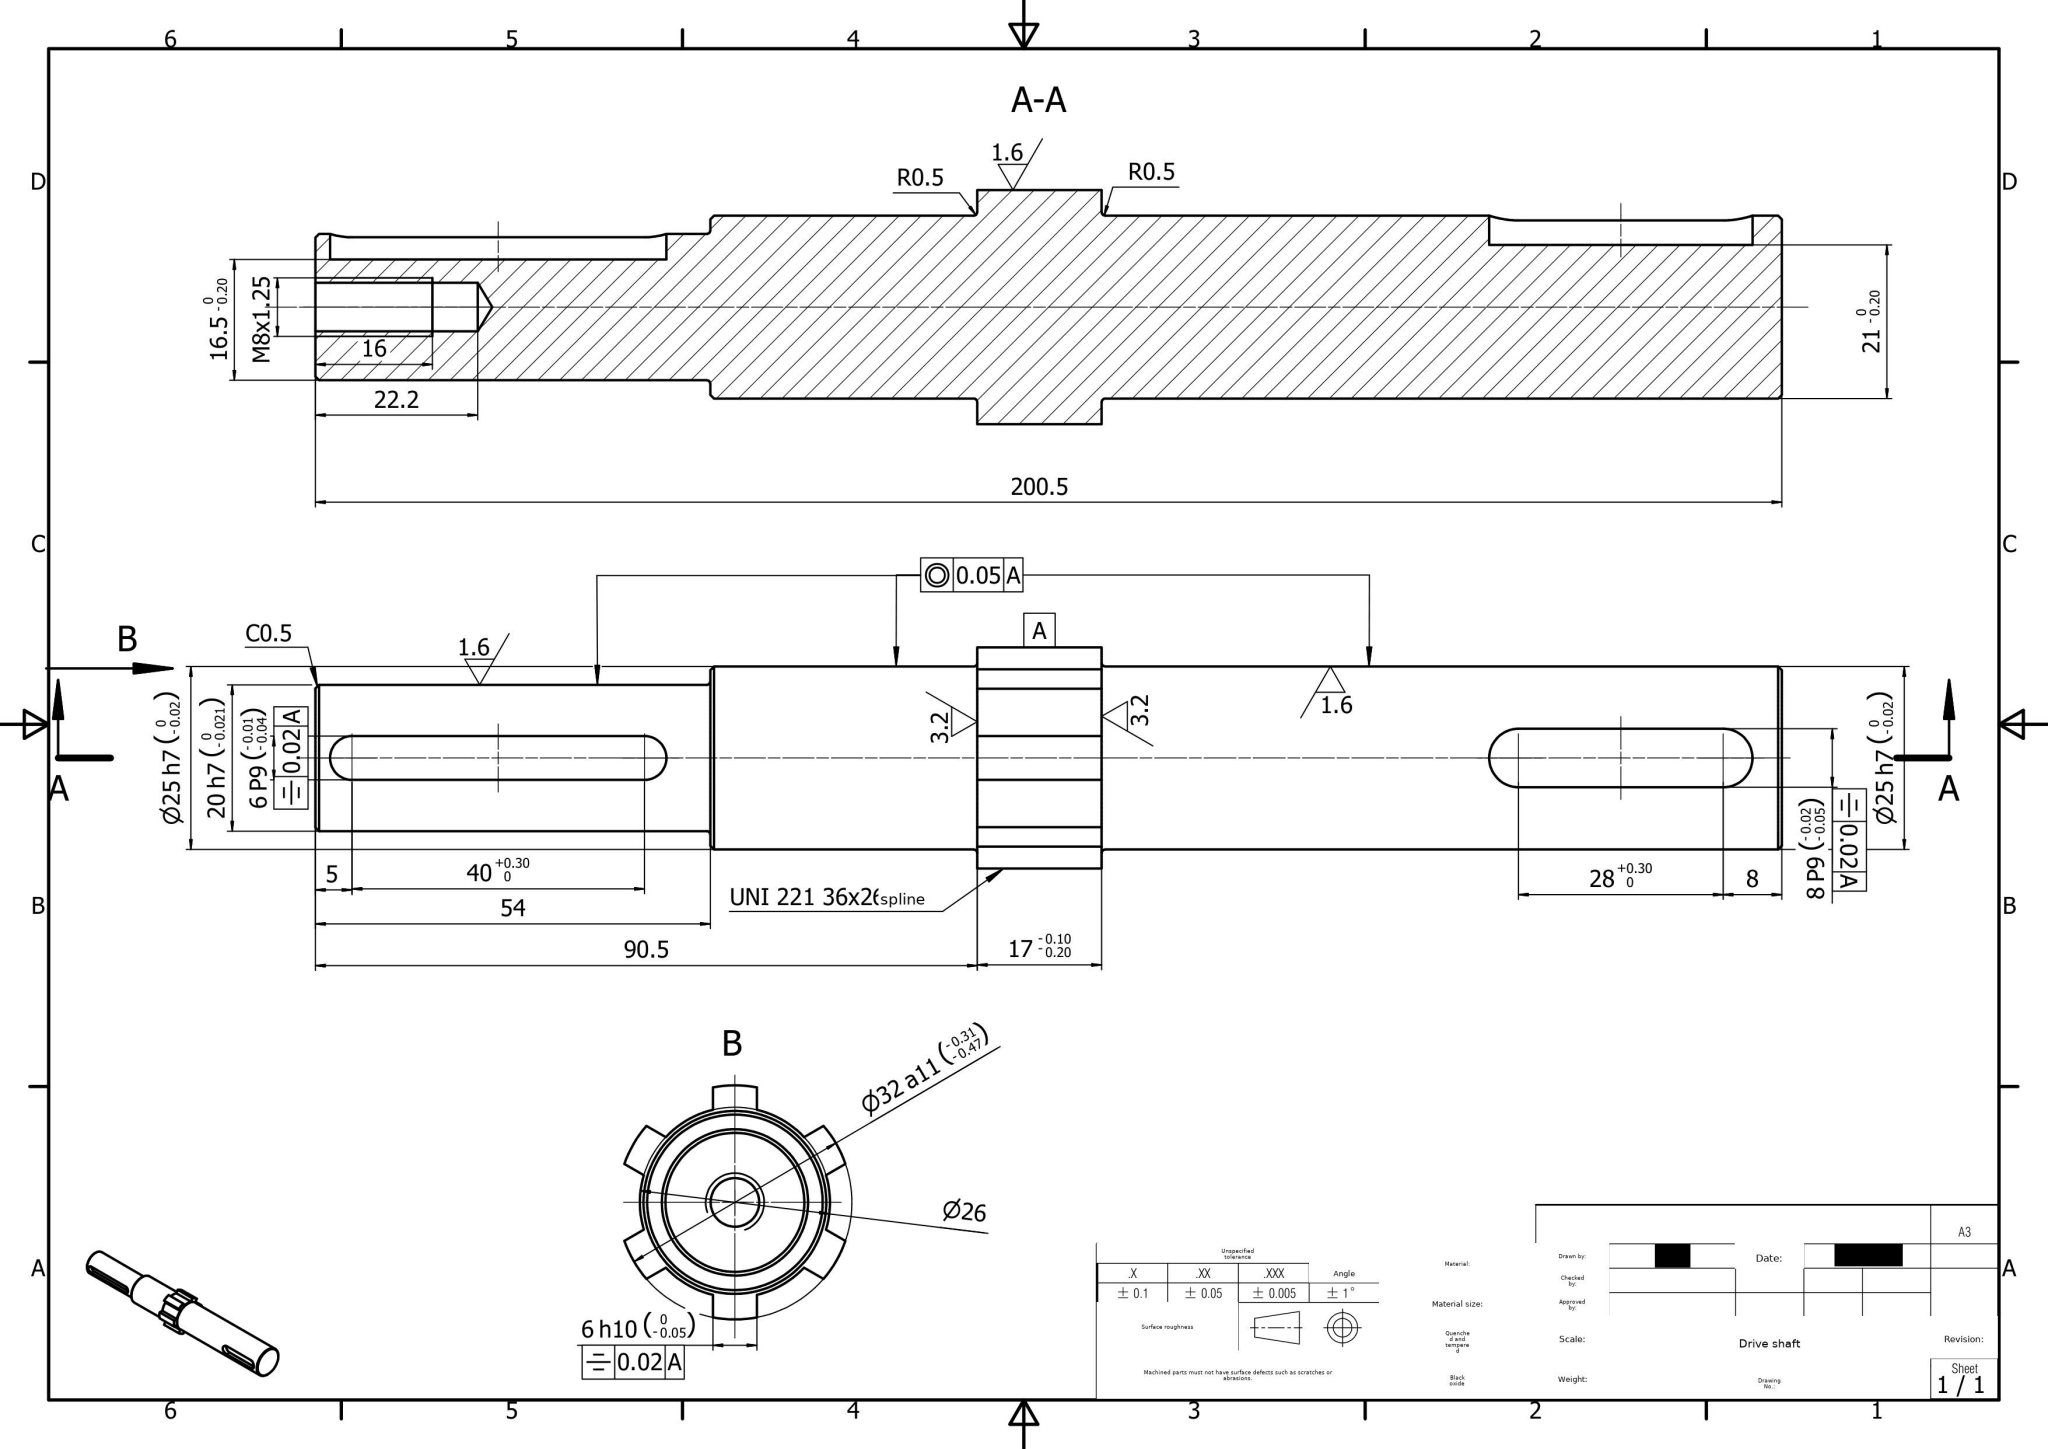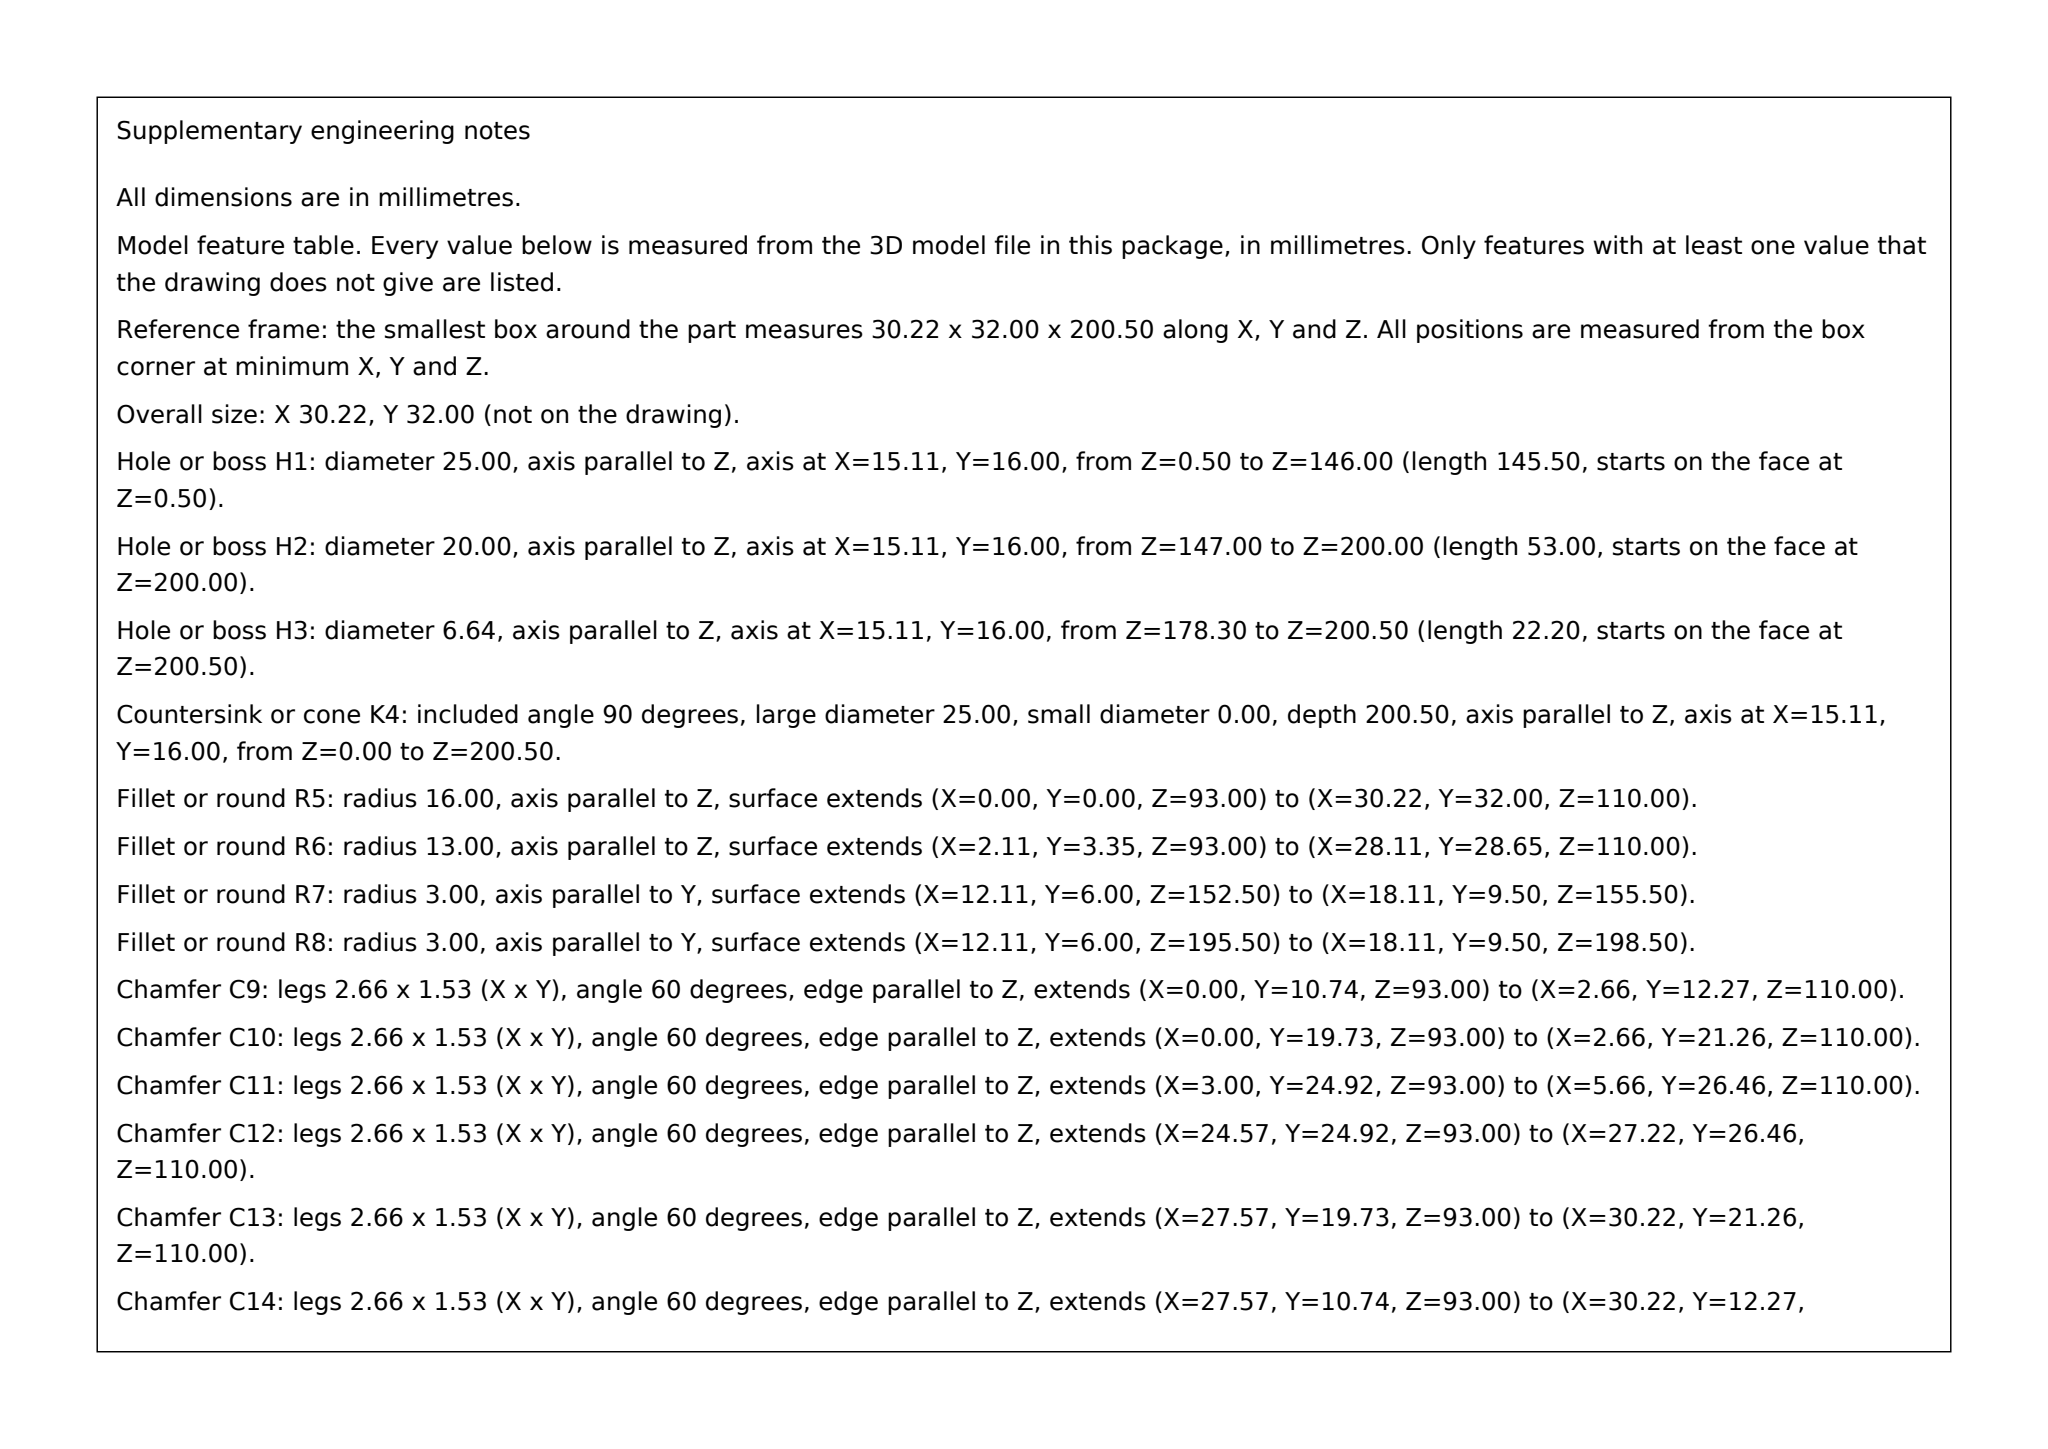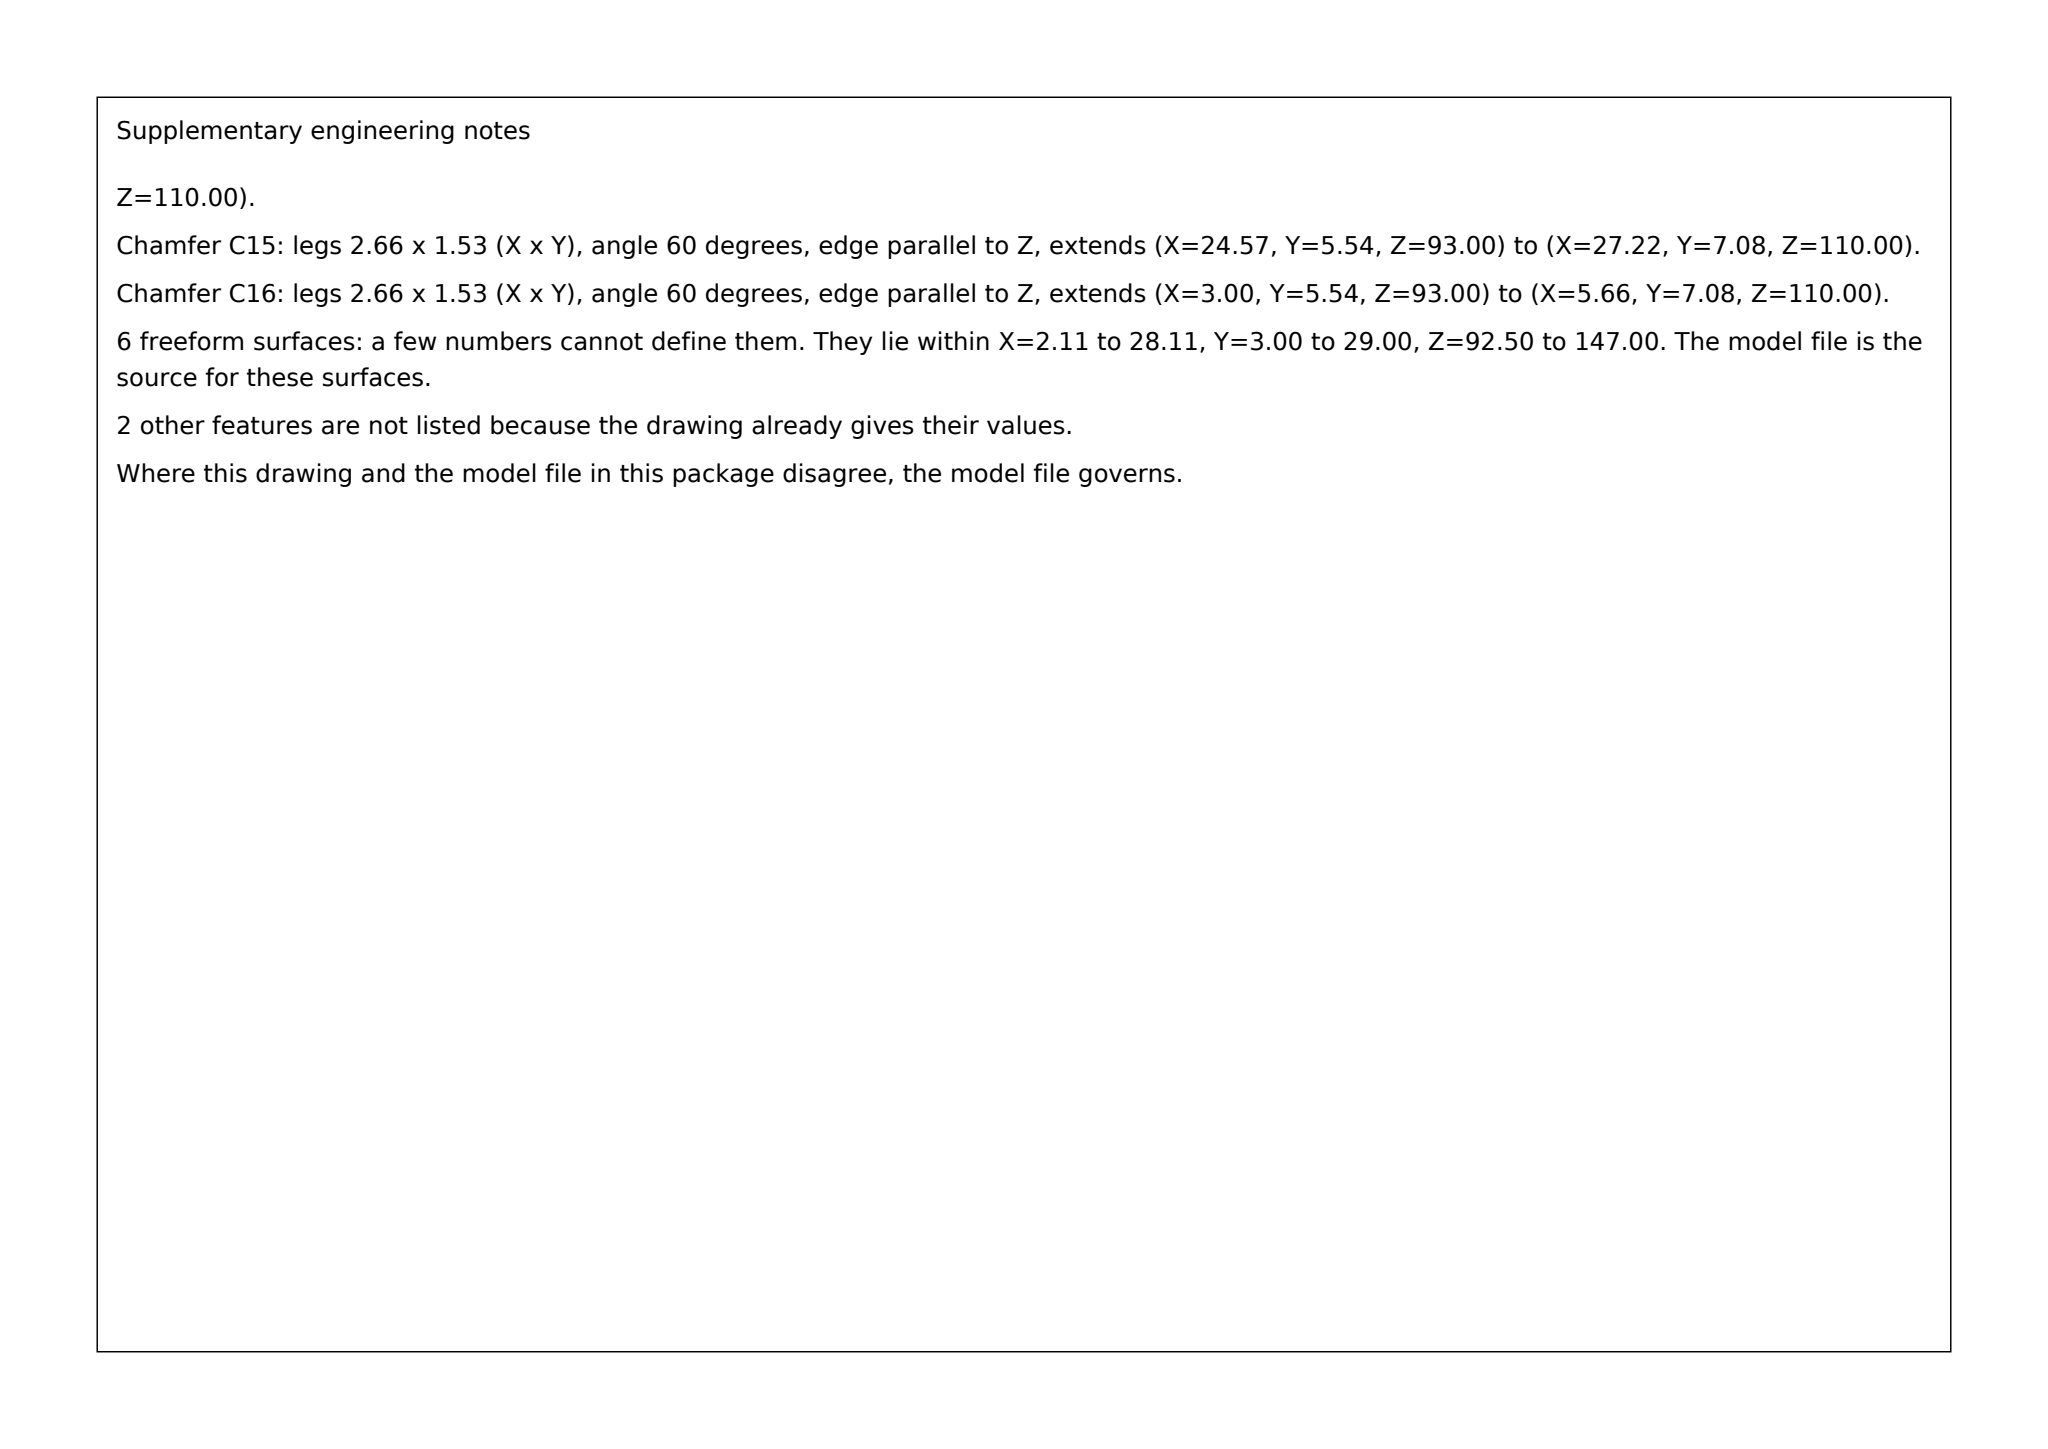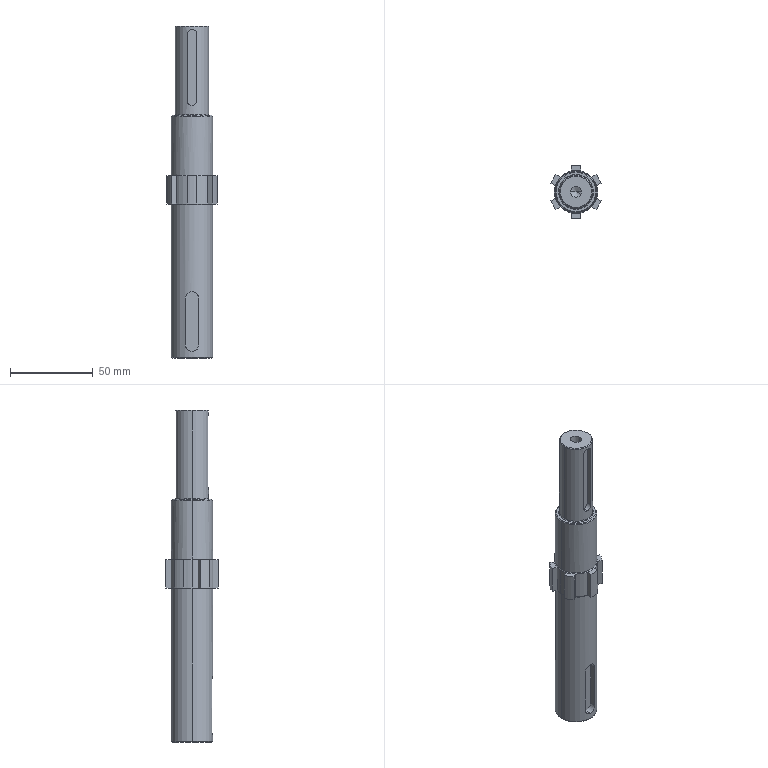Part | SolidWorks | mm | 1 solid | 74 faces | box 30.22 x 32 x 200.5 mm | volume 88663 mm3 | plane 33 | cylinder 27 | cone 8 | spline 6 | commonest cylinder face diameters 26 x7 32 x6 25 x4 8 x3 6 x3 20 x2 6.647 x2